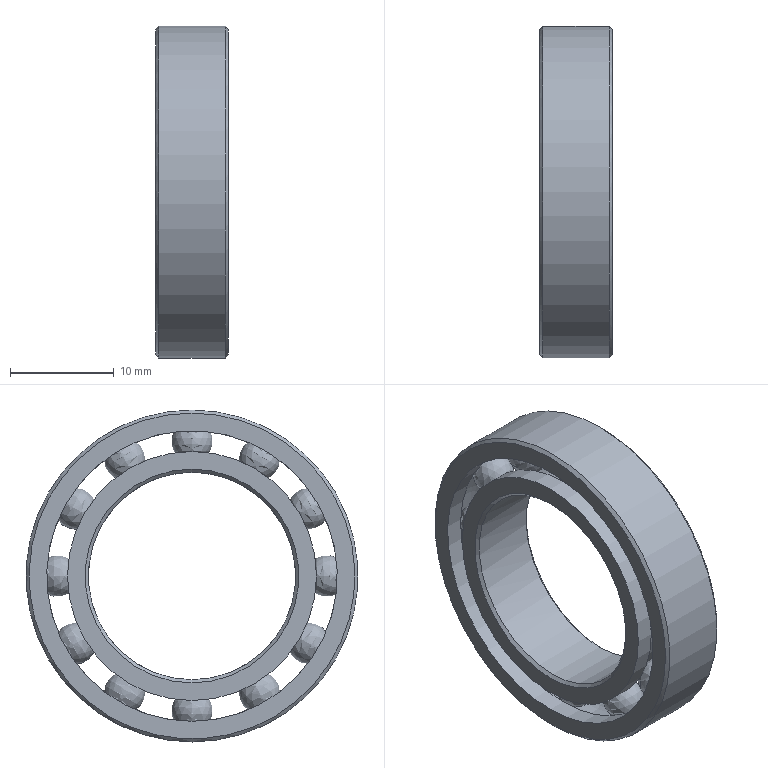Component | NX | GB-T276_60000-1994_61804 | 14 solids | 28 faces | volume 2273 mm3 | sphere 12 | cylinder 6 | plane 4 | cone 4 | torus 2 | commonest cylinder face diameters 28 x2 24 x2 32 x1 20 x1